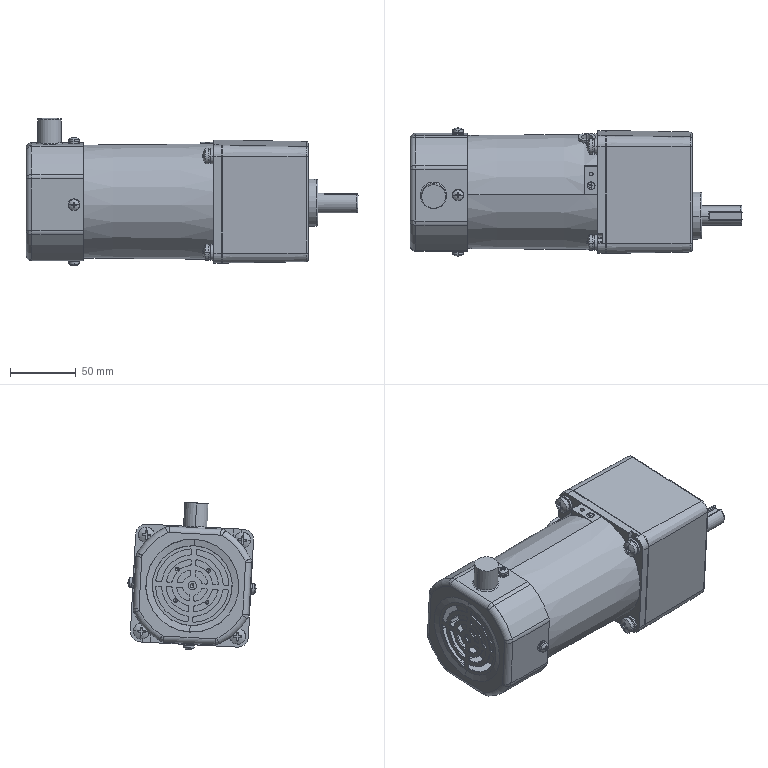Component | SolidWorks | StepperMotor-2 | 28 solids | 856 faces | volume 1251164 mm3 | cylinder 405 | plane 307 | cone 54 | torus 48 | sphere 24 | spline 18 | commonest cylinder face diameters 2 x53 0.6 x32 9 x25 4.3 x24 12 x22 4.4 x16 6.6 x16 4 x16